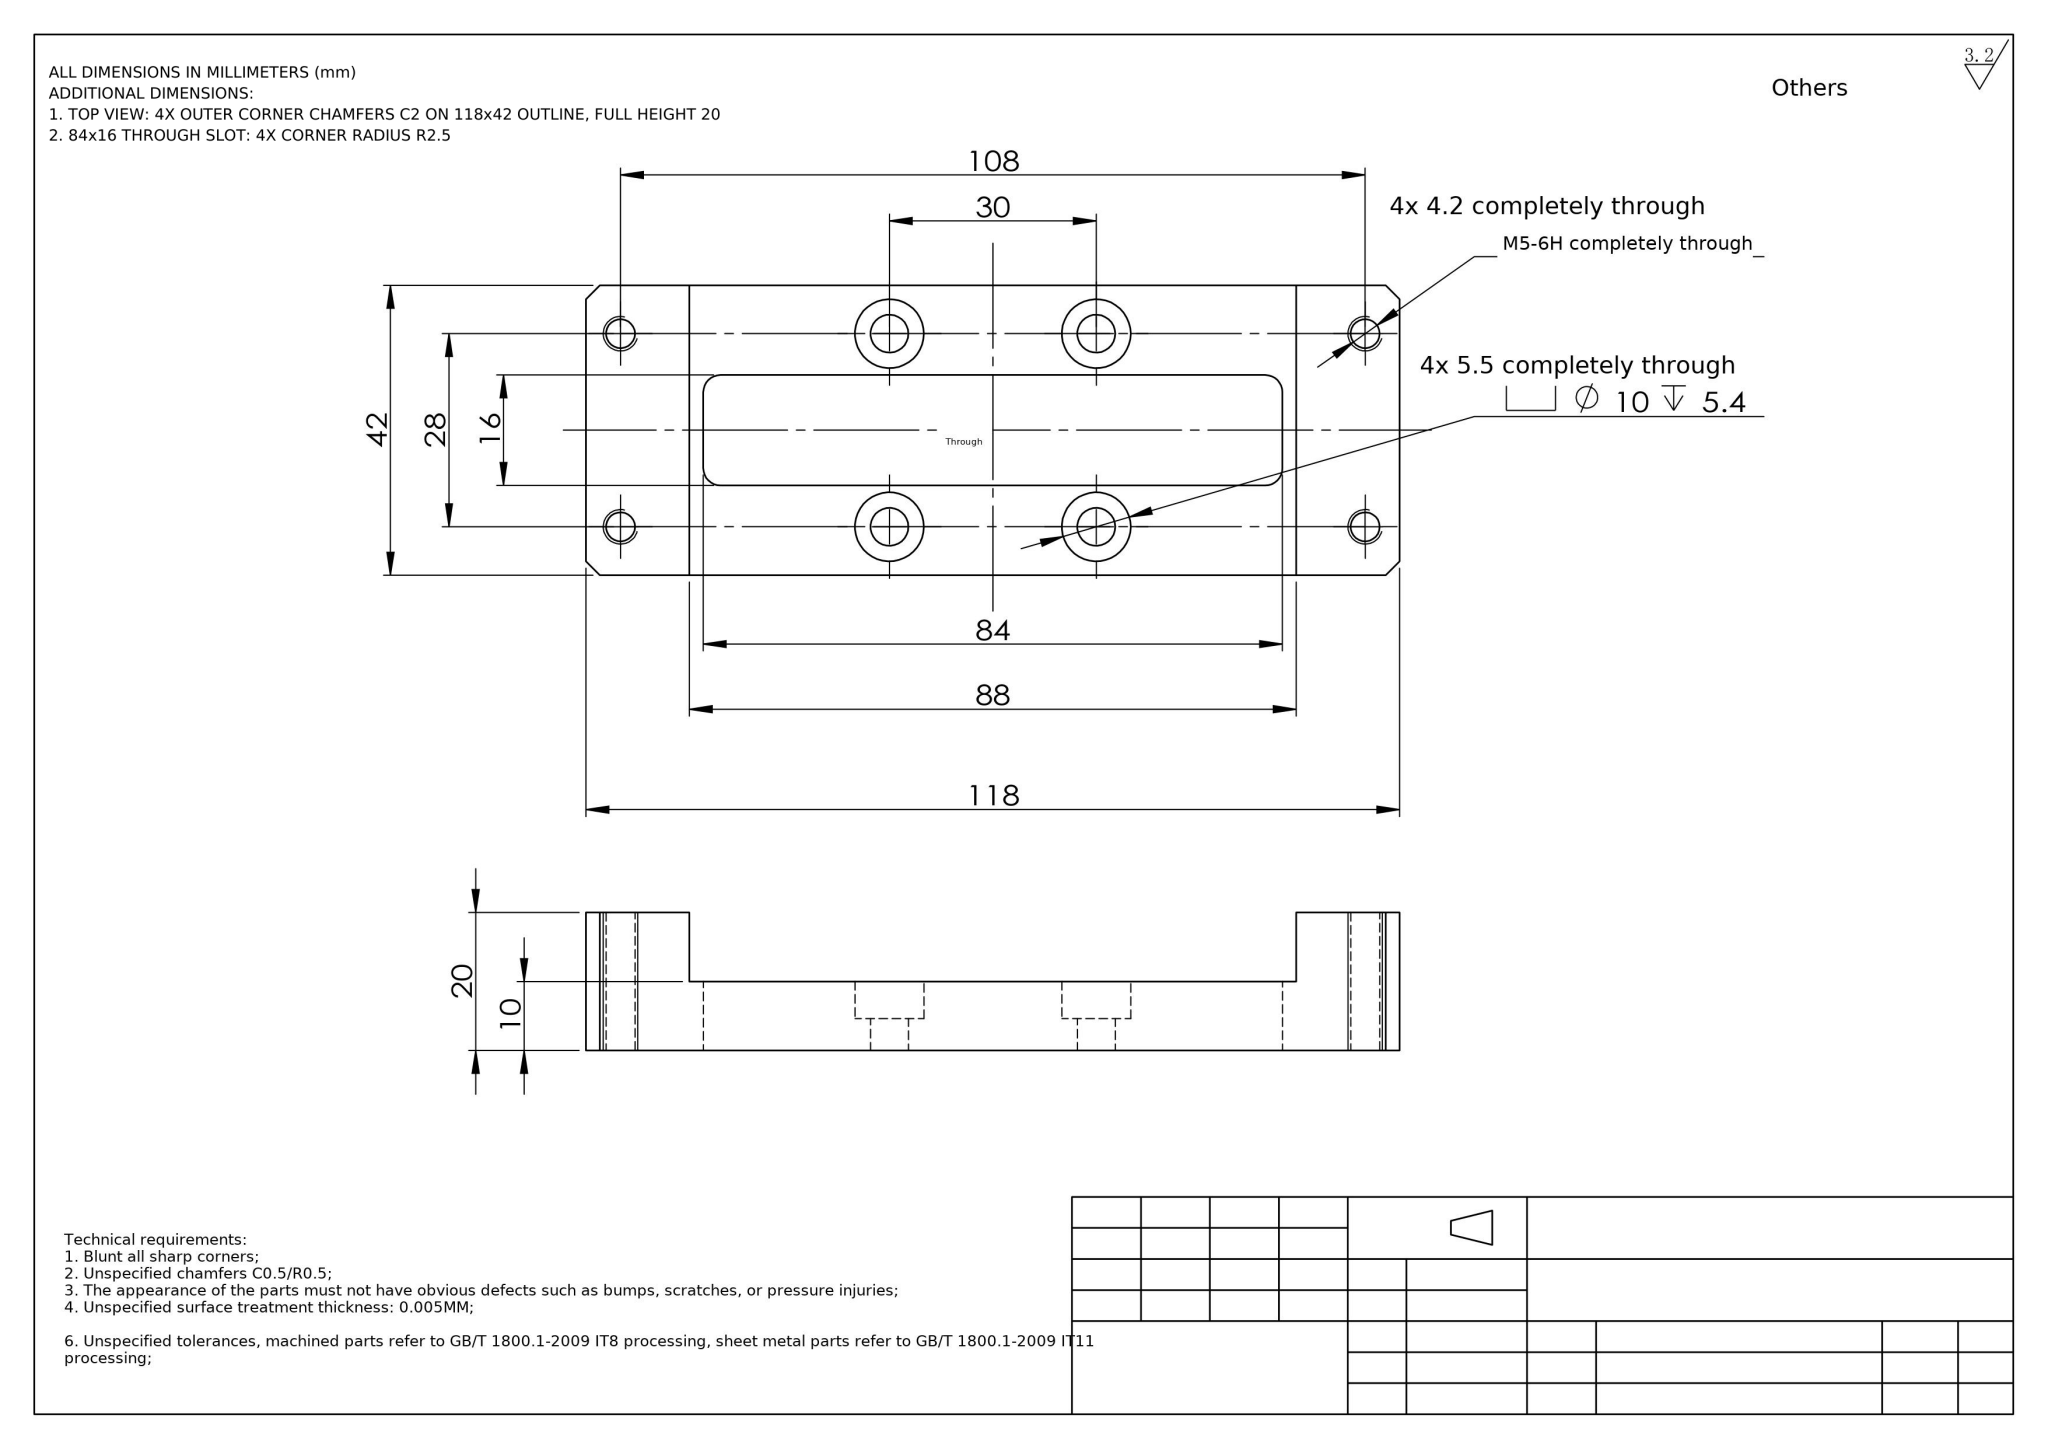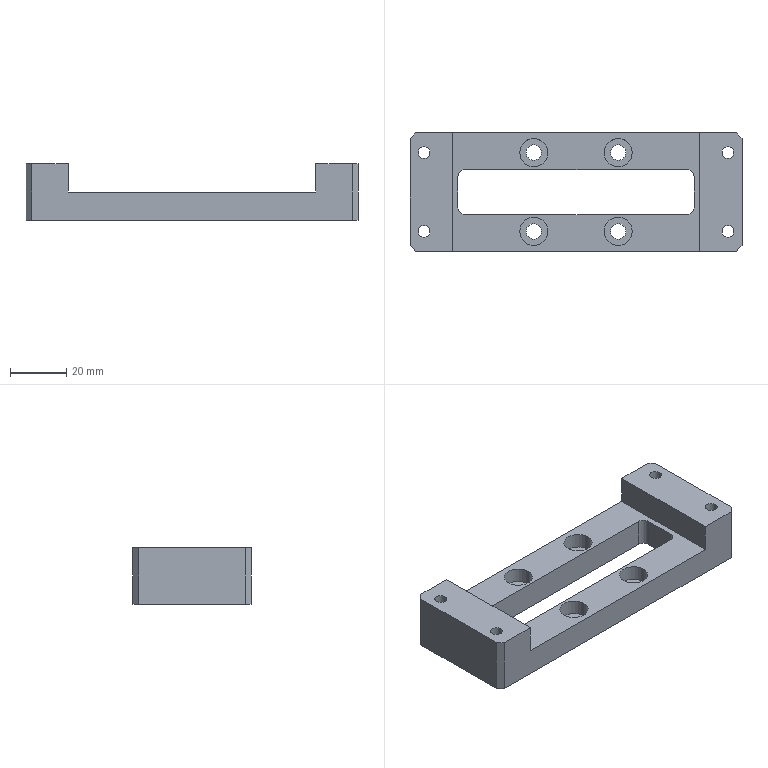Part | NX | mm | 1 solid | 50 faces | box 118 x 42 x 20 mm | volume 45372 mm3 | cylinder 28 | plane 22 | commonest cylinder face diameters 4.2 x8 10 x8 5.5 x8 5 x4